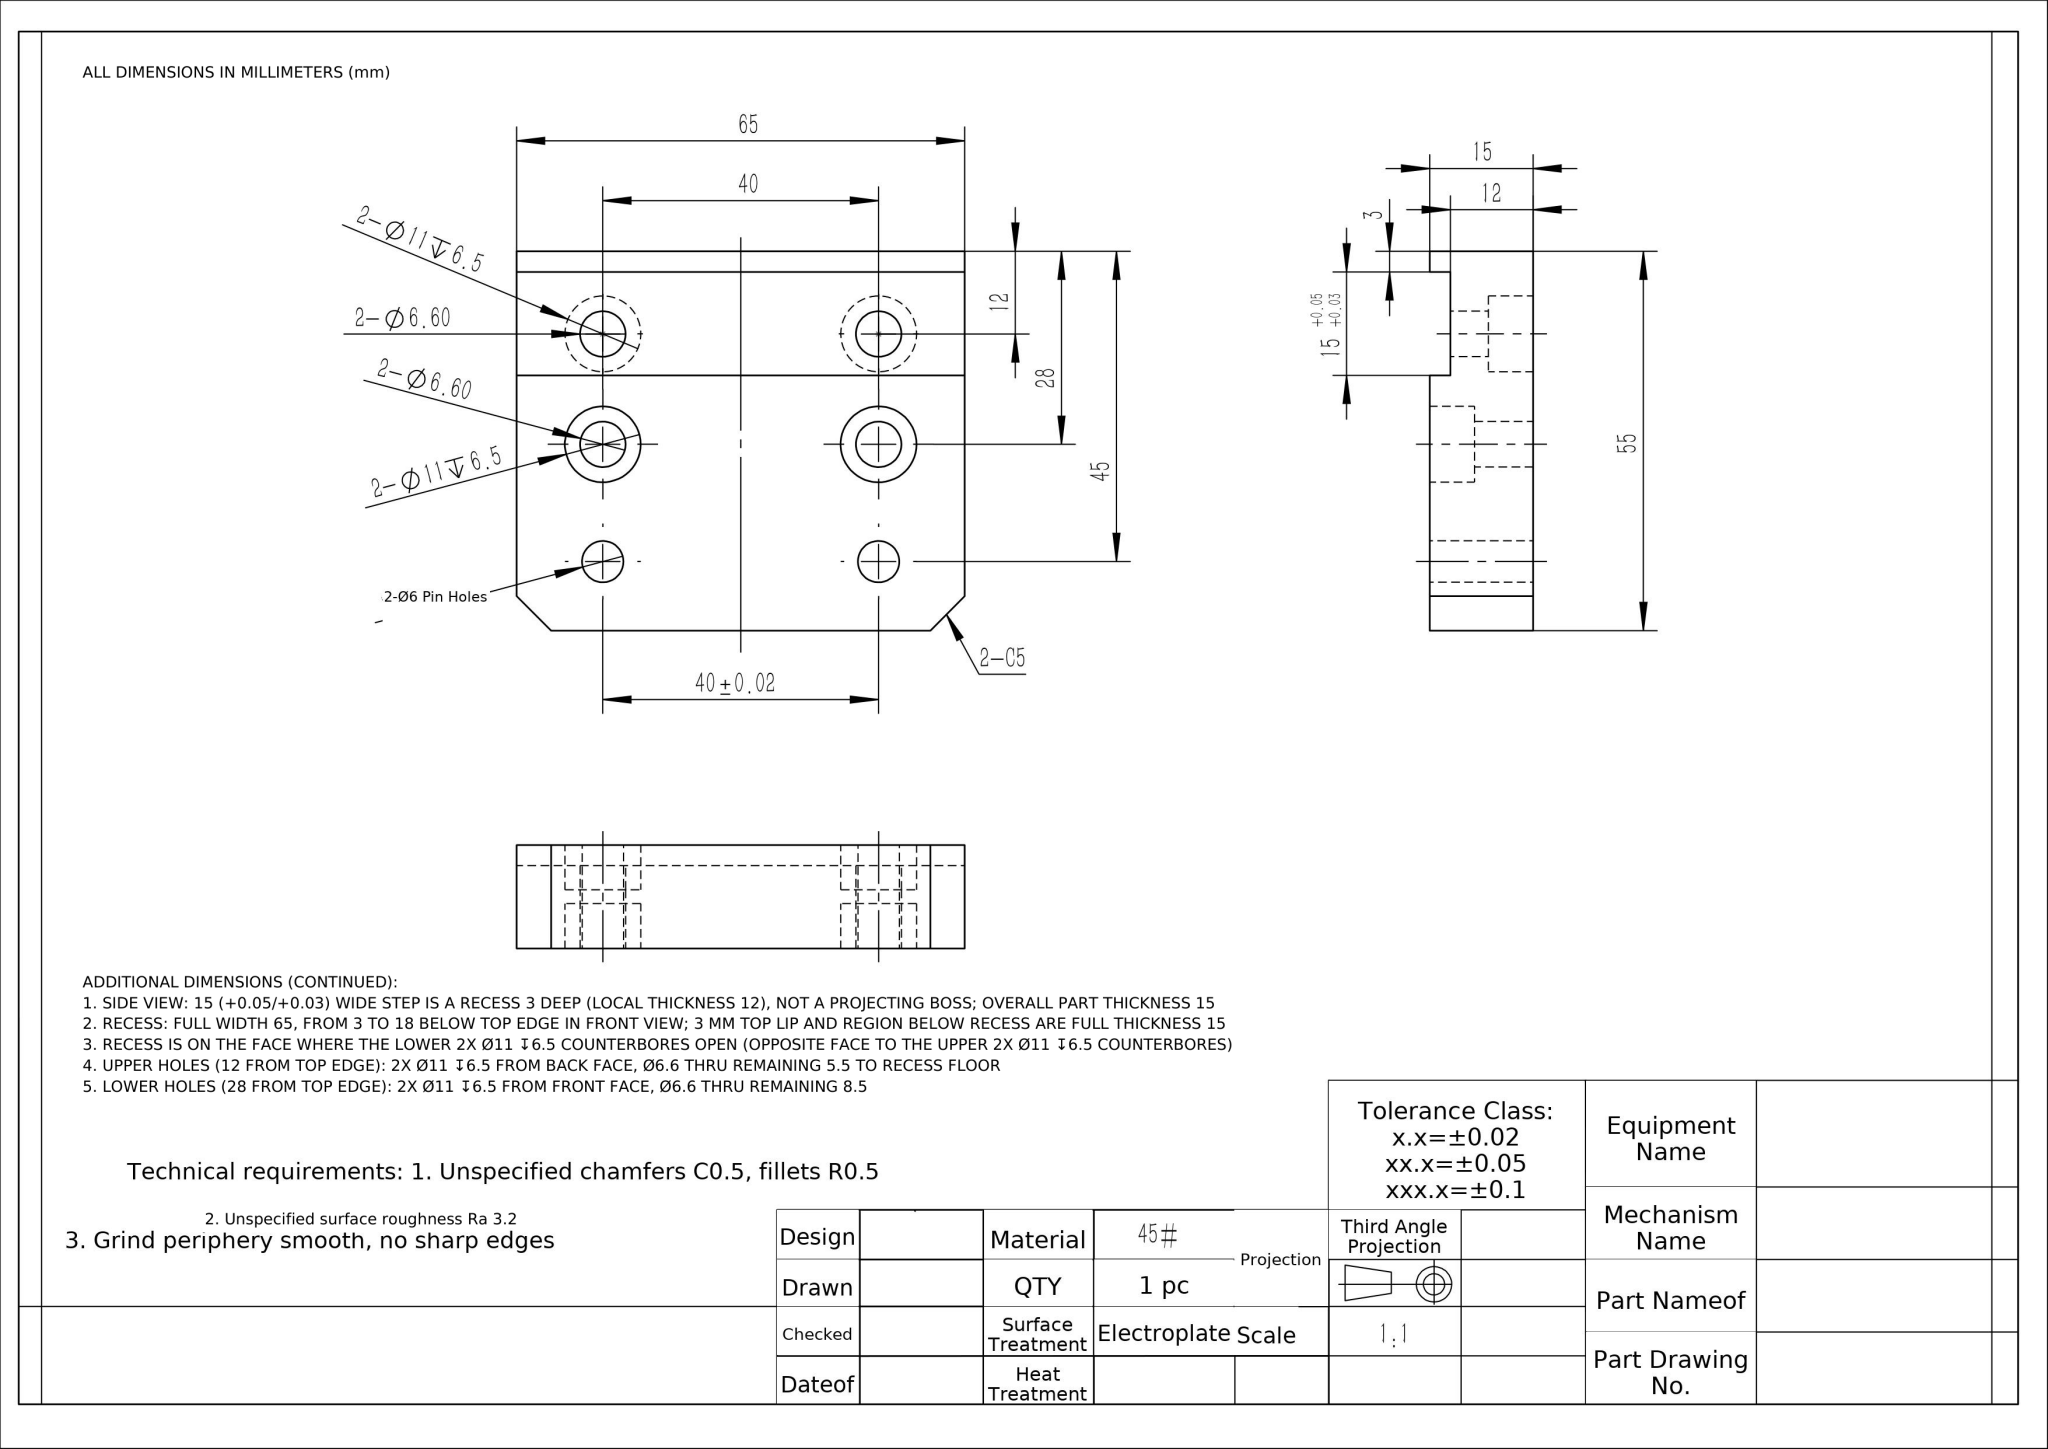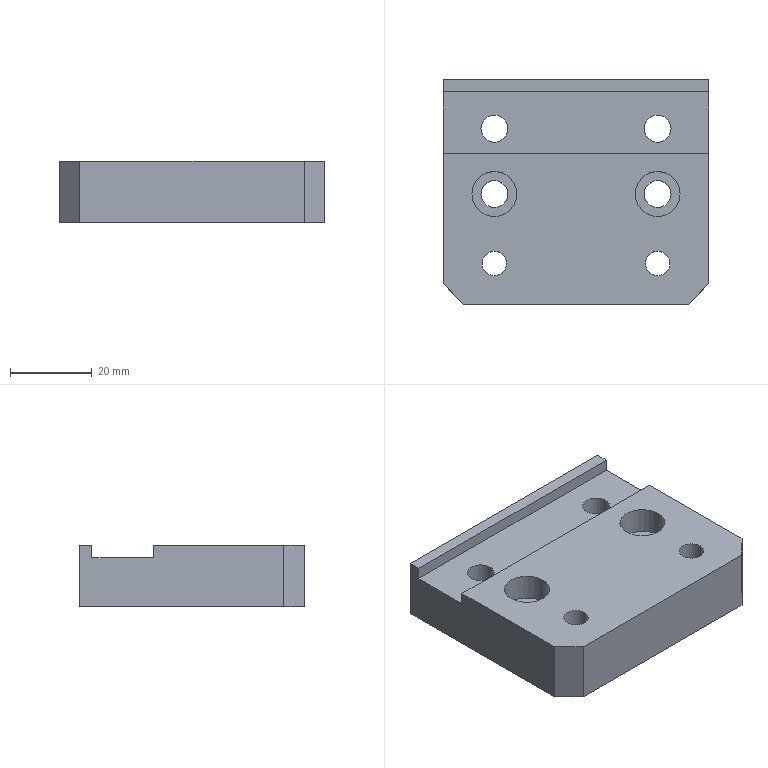Part | NX | mm | 1 solid | 36 faces | box 65 x 55 x 15 mm | volume 46048 mm3 | cylinder 20 | plane 16 | commonest cylinder face diameters 11 x8 6.6 x8 6 x4